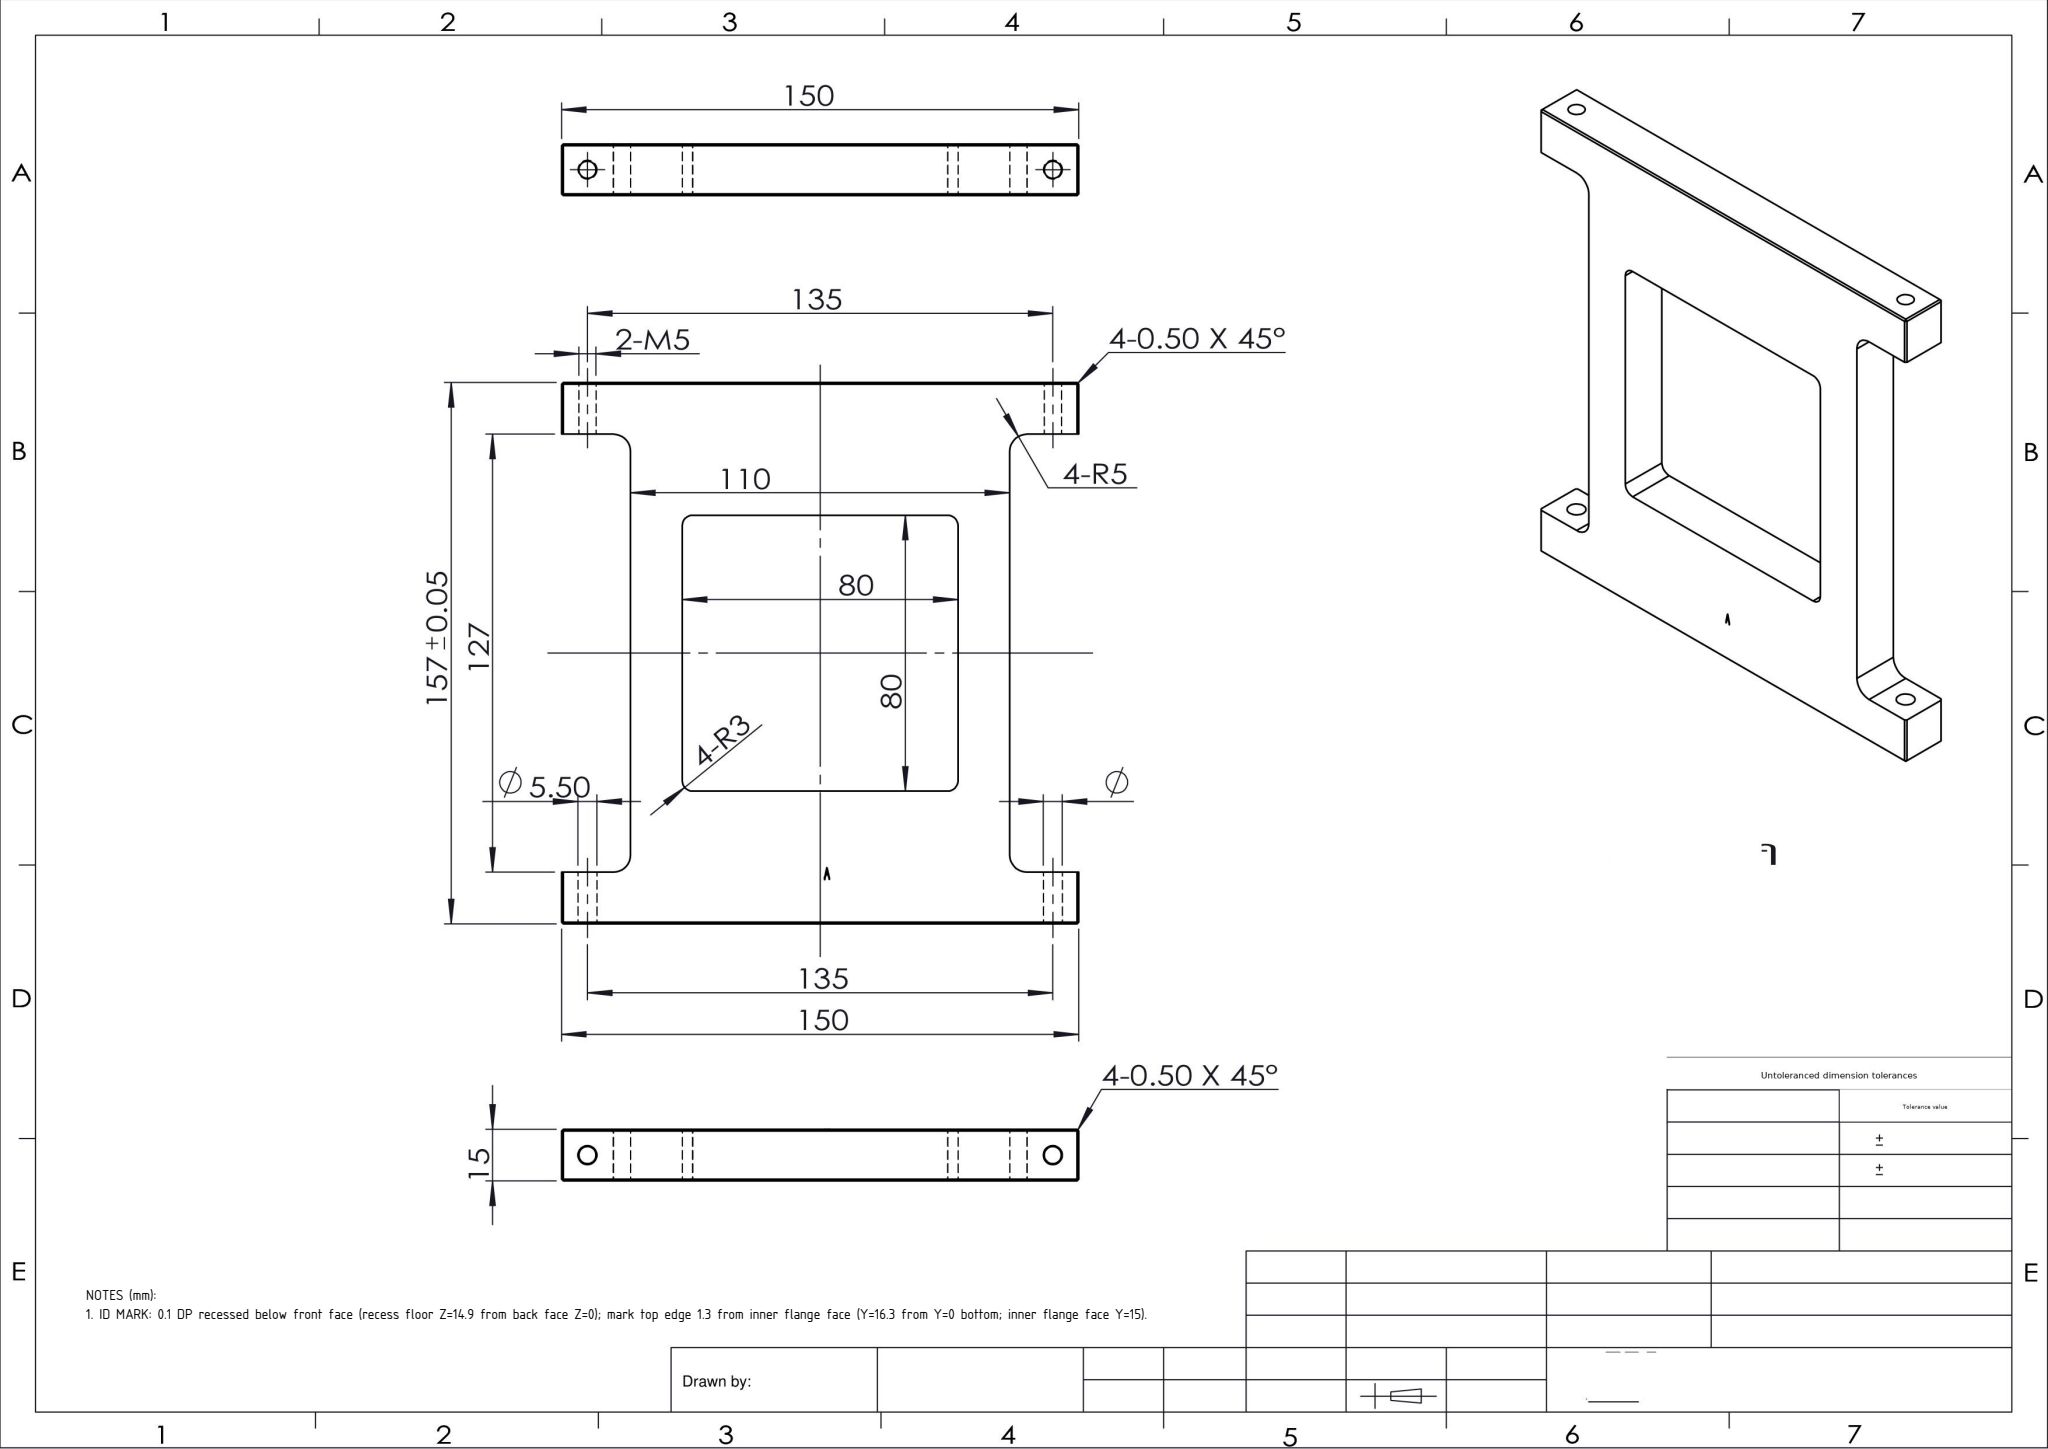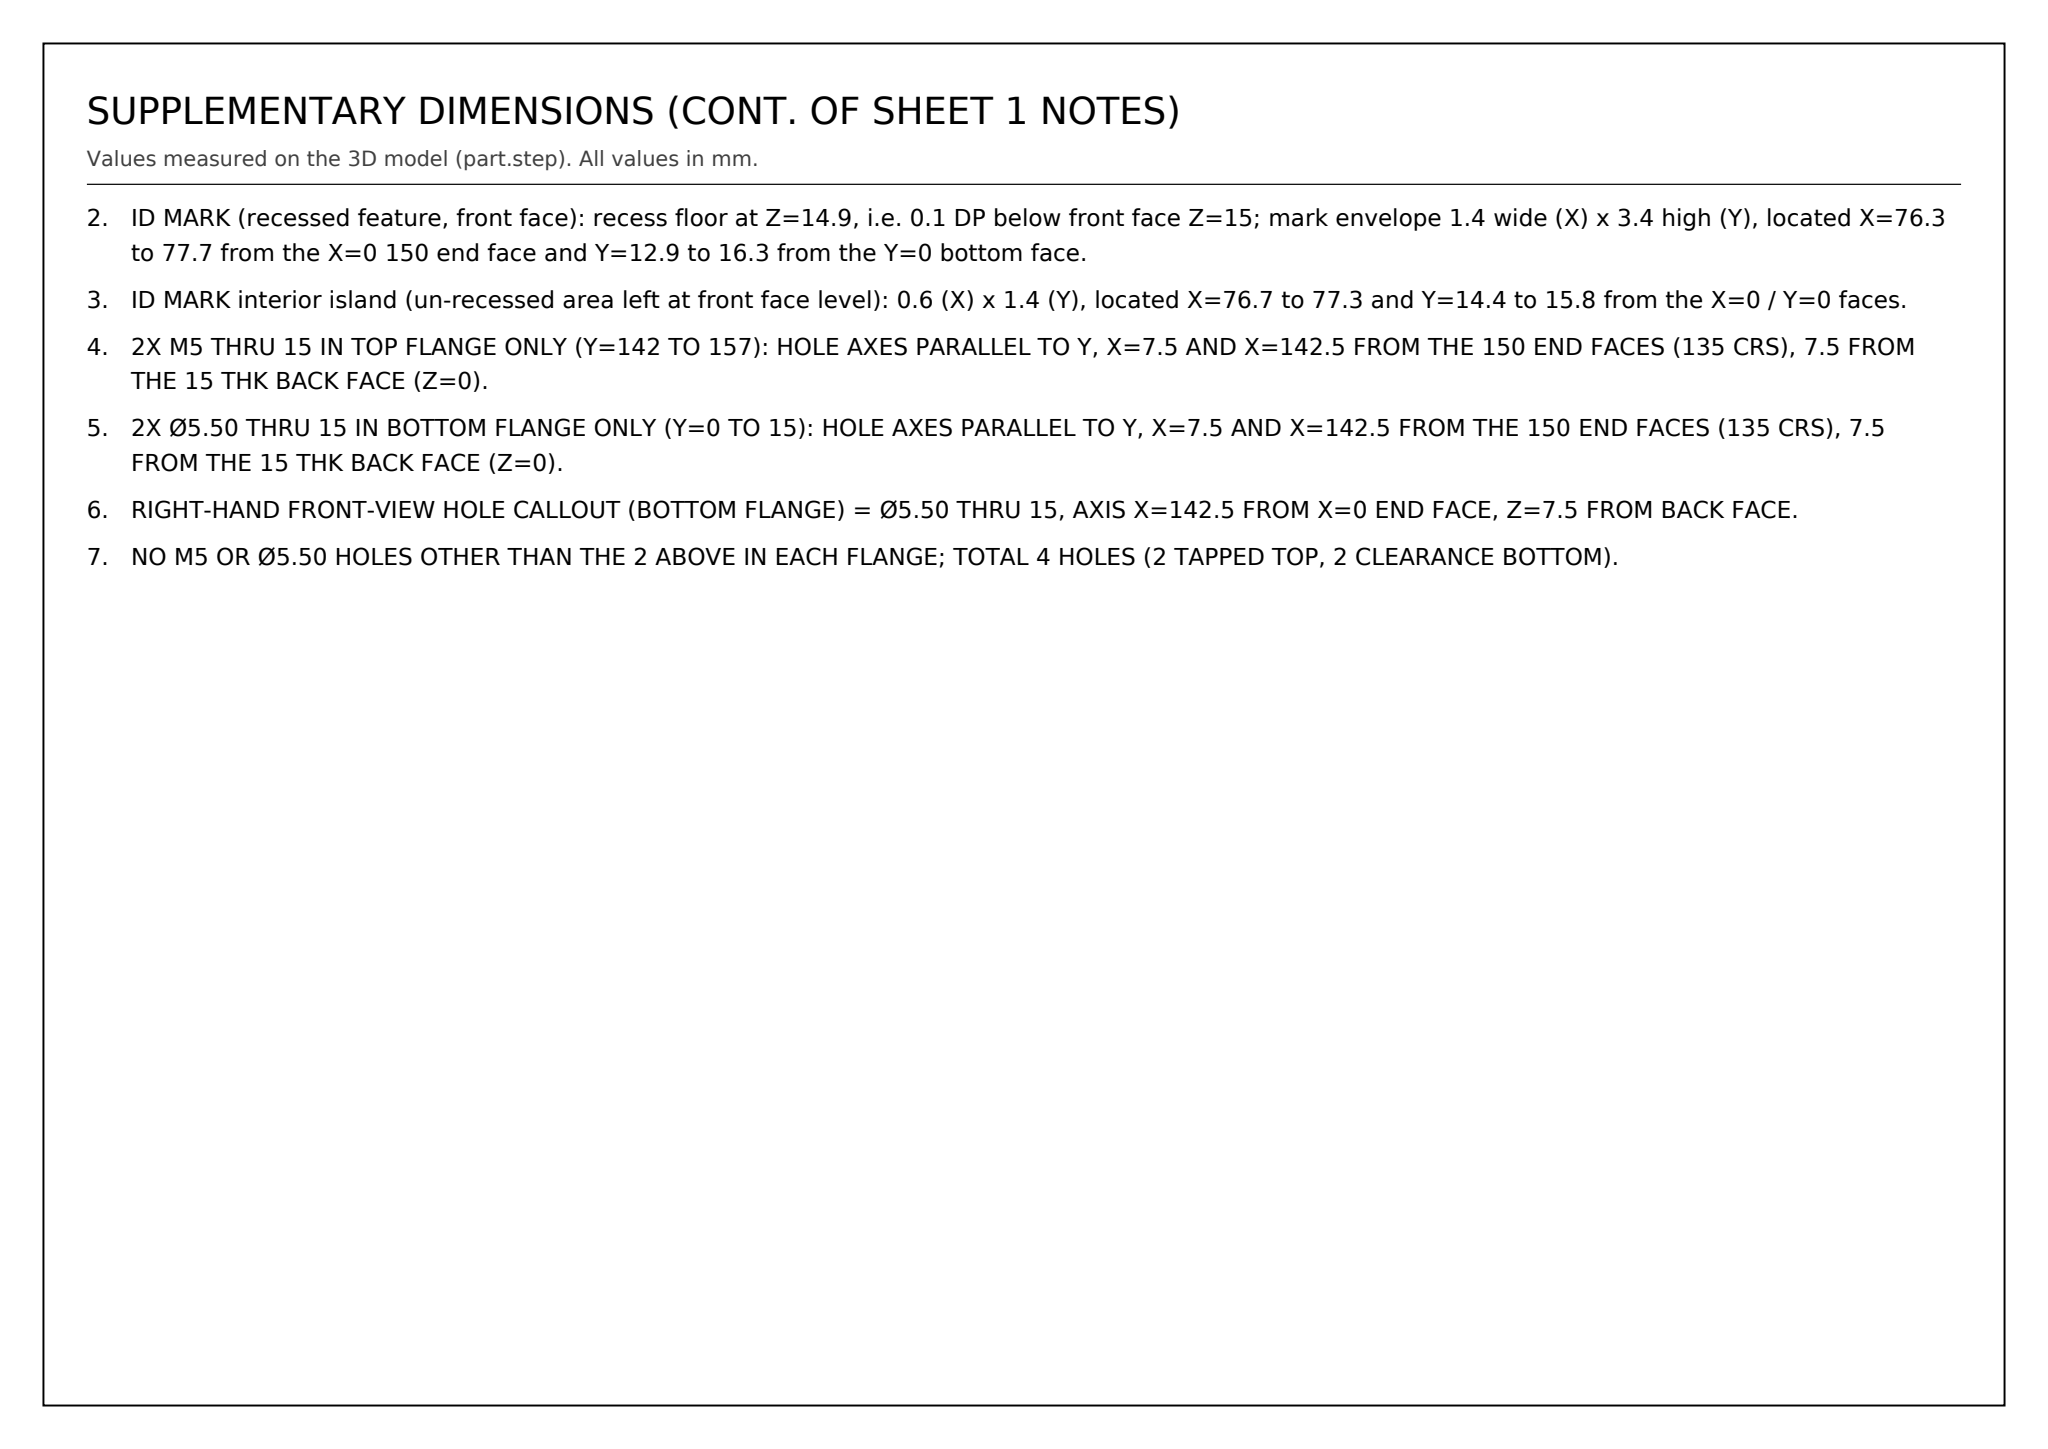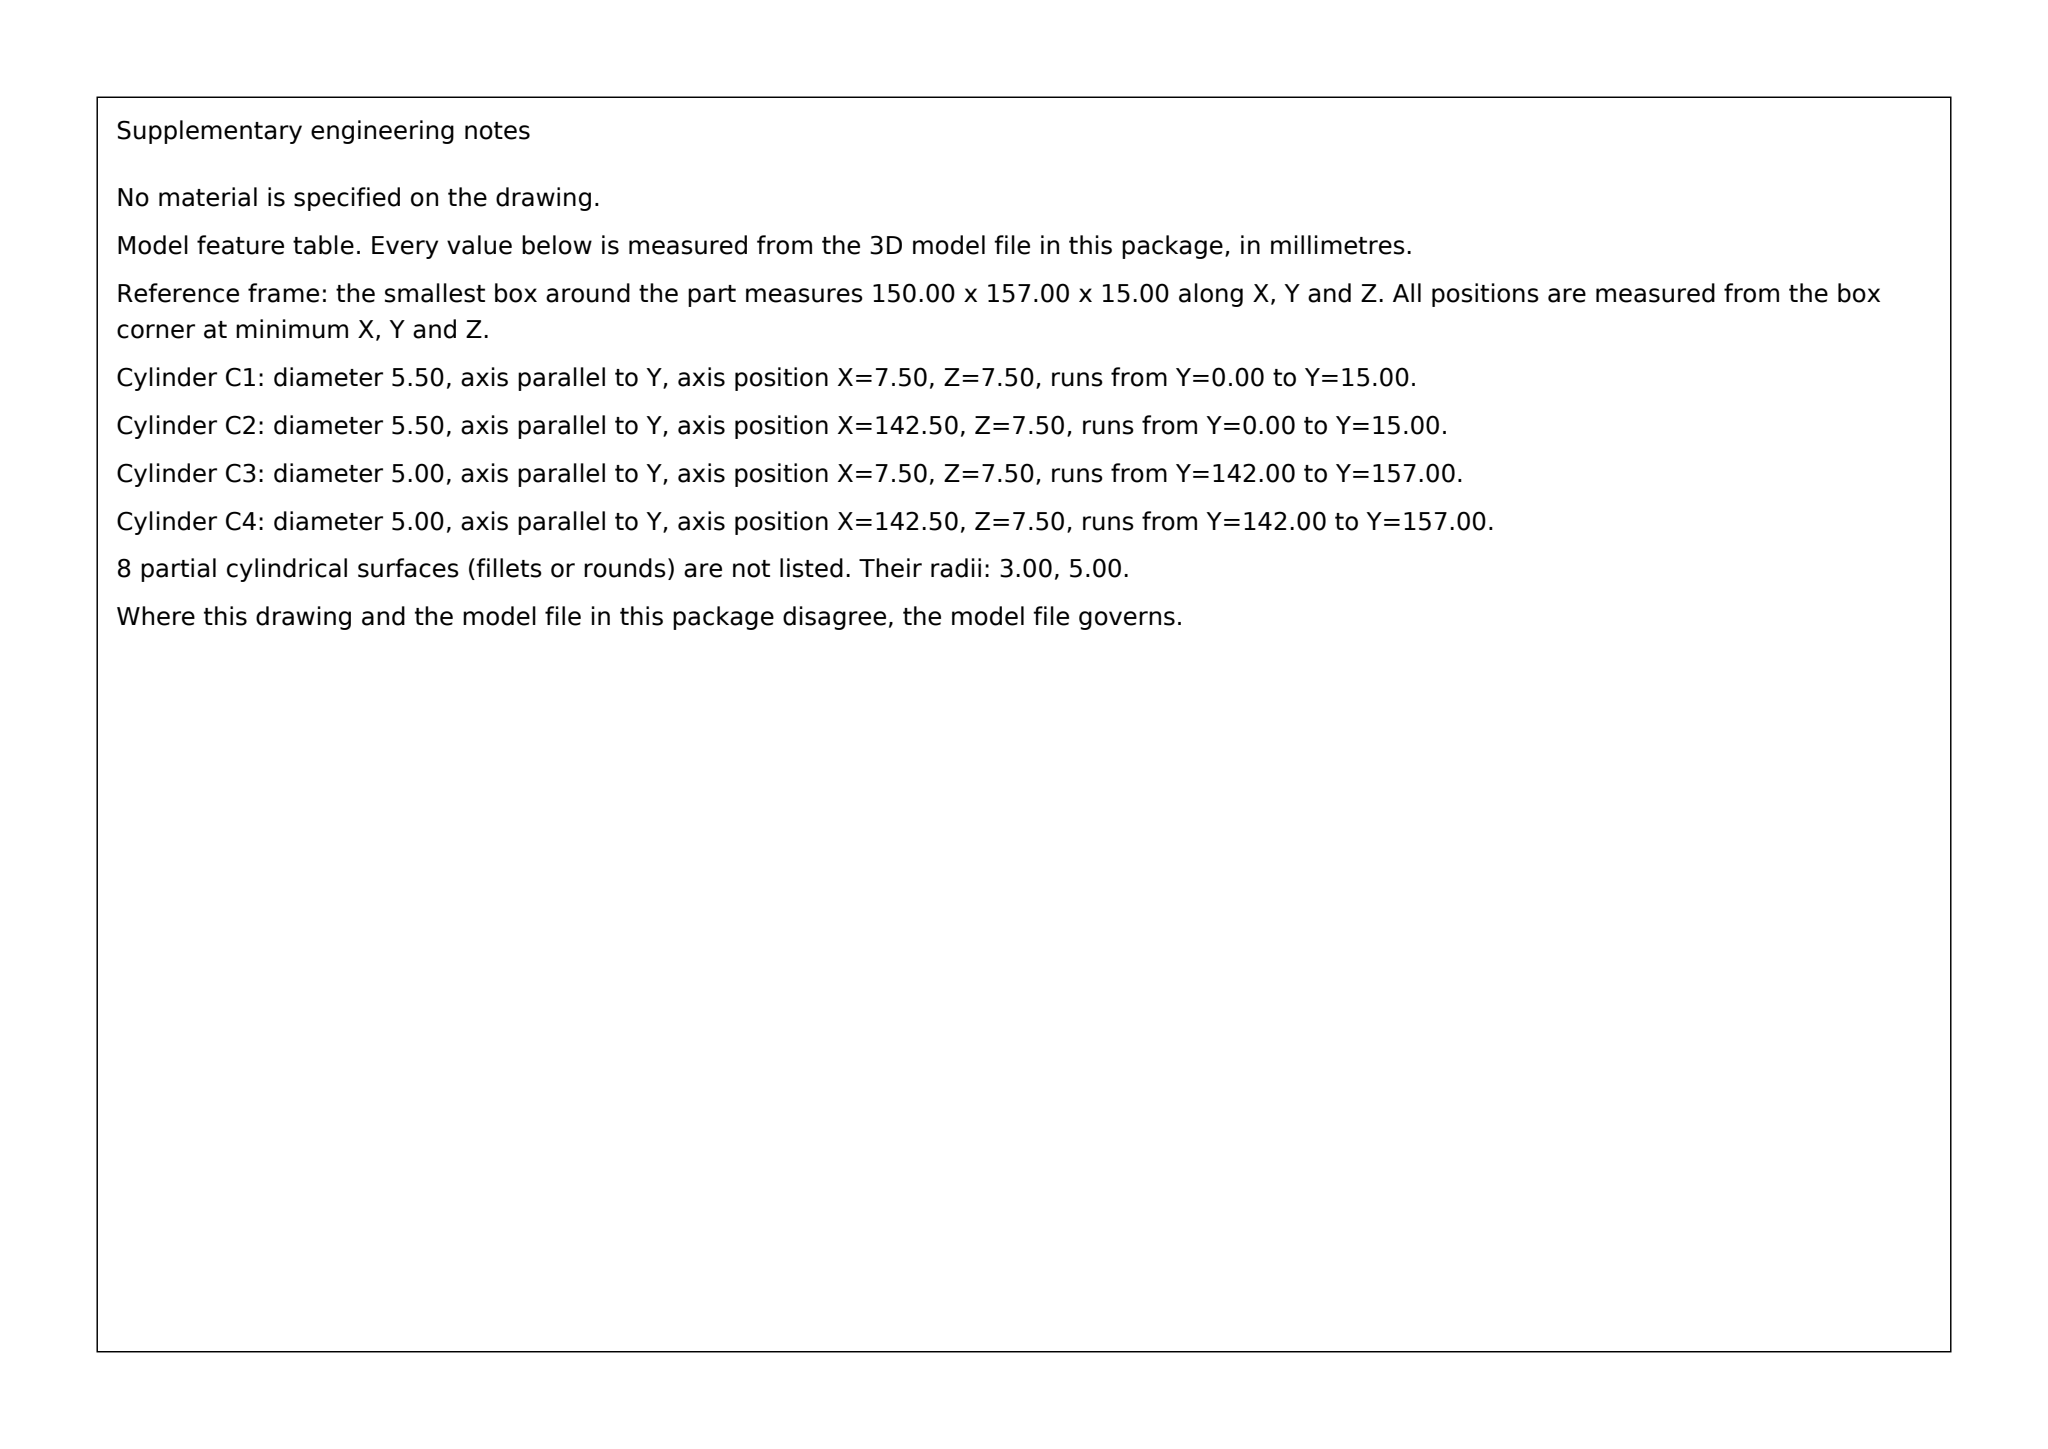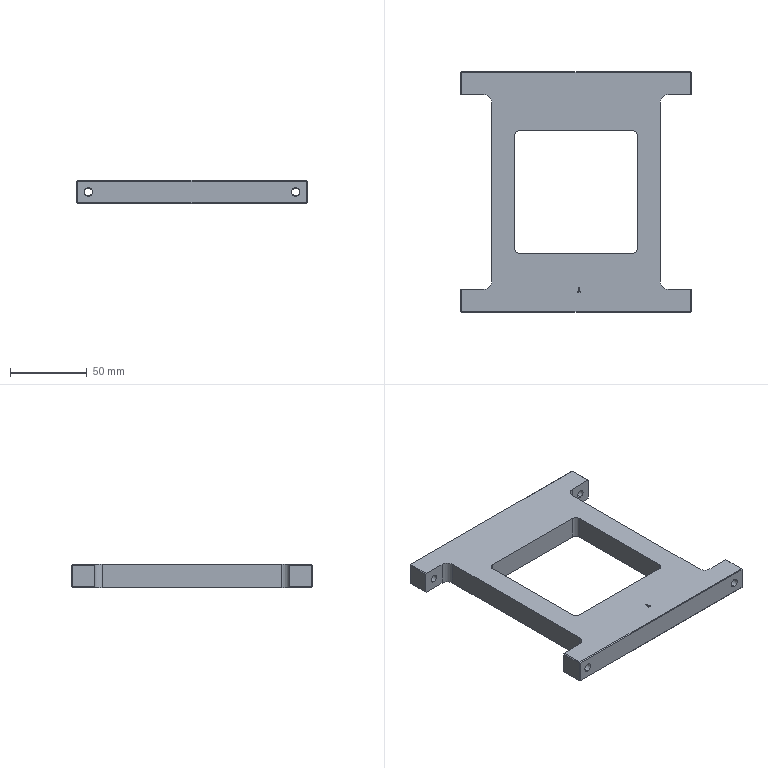Part | SolidWorks | mm | 1 solid | 86 faces | box 150 x 157 x 15 mm | volume 180089 mm3 | plane 63 | cylinder 16 | spline 7 | commonest cylinder face diameters 5.5 x4 5 x4 10 x4 6 x4
Drawing notes:
ID MARK: 0.1 DP recessed below front face (recess floor Z=14.9 from back face Z=0); mark top edge 1.3 from inner flange face (Y=16.3 from Y=0 bottom; inner flange face Y=15). | from the solid: axis_planes: z=14.9 plane x[76.3,77.7] y[12.9,16.3] (0.1 below front face z=15.0); y=16.3 plane at x[76.9,77.0], z[14.9,15.0]; flange inner face y=15.0; 16.3-15.0=1.3
ID MARK (recessed feature, front face): recess floor at Z=14.9, i.e. 0.1 DP below front face Z=15; mark envelope 1.4 wide (X) x 3.4 high (Y), located X=76.3 to 77.7 from the X=0 150 end face and Y=12.9 to 16.3 from the Y=0 bottom face. | from the solid: axis_planes[z, offset 14.9, extent x:[76.3,77.7], y:[12.9,16.3]] and axis_planes[z, offset 15.0] front face
ID MARK interior island (un-recessed area left at front face level): 0.6 (X) x 1.4 (Y), located X=76.7 to 77.3 and Y=14.4 to 15.8 from the X=0 / Y=0 faces. | from the solid: axis_planes[z, offset 15.0, extent x:[76.7,77.3], y:[14.4,15.8]]
2X M5 THRU 15 IN TOP FLANGE ONLY (Y=142 TO 157): HOLE AXES PARALLEL TO Y, X=7.5 AND X=142.5 FROM THE 150 END FACES (135 CRS), 7.5 FROM THE 15 THK BACK FACE (Z=0). | from the solid: cylinders: hole/bore dia 5.0 axis y at (x=7.5,z=7.5) and (x=142.5,z=7.5), from y=142 to y=157
2X Ø5.50 THRU 15 IN BOTTOM FLANGE ONLY (Y=0 TO 15): HOLE AXES PARALLEL TO Y, X=7.5 AND X=142.5 FROM THE 150 END FACES (135 CRS), 7.5 FROM THE 15 THK BACK FACE (Z=0). | from the solid: cylinders: hole/bore dia 5.5 axis y at (x=7.5,z=7.5) and (x=142.5,z=7.5), from y=0 to y=15
RIGHT-HAND FRONT-VIEW HOLE CALLOUT (BOTTOM FLANGE) = Ø5.50 THRU 15, AXIS X=142.5 FROM X=0 END FACE, Z=7.5 FROM BACK FACE. | from the solid: cylinders: hole/bore dia 5.5 axis y at (x=142.5,z=7.5), from y=0 to y=15
NO M5 OR Ø5.50 HOLES OTHER THAN THE 2 ABOVE IN EACH FLANGE; TOTAL 4 HOLES (2 TAPPED TOP, 2 CLEARANCE BOTTOM). | from the solid: cylinders list contains only 4 full 360° hole/bore entries (2X dia 5.0, 2X dia 5.5)
build123d program:
from build123d import *

# Parameters (mm, degrees)
SKETCH1_W           = 150
SKETCH1_H           = 157
BOSS_EXTRUDE1_DEPTH = 7.5
SKETCH2_R           = 2.5
CUT_EXTRUDE1_DEPTH  = 20
SKETCH3_W           = 20
SKETCH3_H           = 127
CUT_EXTRUDE2_DEPTH  = 110.6
FILLET1_R           = 5
CHAMFER1_SIZE       = 0.5
SKETCH5_W           = 80
SKETCH5_H           = 80
CUT_EXTRUDE4_DEPTH  = 110.6
FILLET2_R           = 3
CUT_EXTRUDE5_DEPTH  = 0.1
SKETCH7_R           = 2.75
CUT_EXTRUDE6_DEPTH  = 20


with BuildPart() as part:
    # Sketch1 → Boss-Extrude1 (new, symmetric)
    with BuildSketch(Plane.XY):
        Rectangle(SKETCH1_W, SKETCH1_H)
    extrude(amount=BOSS_EXTRUDE1_DEPTH, both=True)

    # Sketch2 → Cut-Extrude1 (cut)
    with BuildSketch(Plane(origin=(0, 78.5, 0), x_dir=(1, 0, 0), z_dir=(0, 1, 0))):
        with Locations(Location((-67.5, 0, 0), (0, 0, 270))):
            Circle(SKETCH2_R)
        with Locations(Location((67.5, 0, 0), (0, 0, 90))):
            Circle(SKETCH2_R)
    extrude(amount=-CUT_EXTRUDE1_DEPTH, mode=Mode.SUBTRACT)

    # Sketch3 → Cut-Extrude2 (cut, through all)
    with BuildSketch(Plane(origin=(0, 0, -7.5), x_dir=(-1, 0, 0), z_dir=(0, 0, -1))):
        with Locations((-65, 0)):
            Rectangle(SKETCH3_W, SKETCH3_H)
        with Locations((65, 0)):
            Rectangle(SKETCH3_W, SKETCH3_H)
    extrude(amount=-CUT_EXTRUDE2_DEPTH, mode=Mode.SUBTRACT)

    # Fillet1
    fillet1_edges = [part.edges().sort_by_distance(p)[0] for p in [
        (55, 63.5, 0),
        (55, -63.5, 0),
        (-55, 63.5, 0),
        (-55, -63.5, 0),
    ]]
    fillet(fillet1_edges, radius=FILLET1_R)

    # Chamfer1
    chamfer1_edges = [part.edges().sort_by_distance(p)[0] for p in [
        (-75, 71, 7.5),
        (0, -78.5, 7.5),
        (75, 71, -7.5),
        (75, 71, 7.5),
        (-75, -71, -7.5),
        (-75, -71, 7.5),
        (75, -71, 7.5),
        (0, -78.5, -7.5),
        (-75, 71, -7.5),
        (0, 78.5, -7.5),
        (75, -71, -7.5),
        (0, 78.5, 7.5),
        (75, -78.5, 0),
        (-75, -78.5, 0),
        (-75, 78.5, 0),
        (75, 78.5, 0),
    ]]
    chamfer(chamfer1_edges, length=CHAMFER1_SIZE)

    # Sketch5 → Cut-Extrude4 (cut, through all)
    with BuildSketch(Plane.XY.offset(7.5)):
        Rectangle(SKETCH5_W, SKETCH5_H)
    extrude(amount=-CUT_EXTRUDE4_DEPTH, mode=Mode.SUBTRACT)

    # Fillet2
    fillet2_edges = [part.edges().sort_by_distance(p)[0] for p in [
        (-40, -40, 0),
        (-40, 40, 0),
        (40, 40, 0),
        (40, -40, 0),
    ]]
    fillet(fillet2_edges, radius=FILLET2_R)

    # Sketch6 → Cut-Extrude5 (cut)
    with BuildSketch(Plane.XY.offset(7.5)):
        with BuildLine():
            Line((2.312, -64.158), (1.627, -64.324))
            Line((1.627, -64.324), (1.466, -65.074))
            Line((1.466, -65.074), (1.39, -65.457))
            Line((1.39, -65.457), (1.36, -65.578))
            add(Edge.make_bspline(
                [(1.36, -65.578), (1.357, -65.586), (1.352, -65.601), (1.342, -65.618), (1.331, -65.626), (1.318, -65.628), (1.309, -65.617), (1.304, -65.604), (1.302, -65.584), (1.297, -65.558), (1.295, -65.521), (1.291, -65.493), (1.289, -65.477)],
                knots=[0, 0, 0, 0, 1.227, 2.069, 2.596, 3.064, 3.56, 4.322, 5.03, 6.209, 7.852, 10, 10, 10, 10], degree=3))
            Line((1.289, -65.477), (1.265, -65.266))
            add(Edge.make_bspline(
                [(1.265, -65.266), (1.263, -65.249), (1.26, -65.218), (1.258, -65.176), (1.258, -65.147), (1.259, -65.122), (1.267, -65.099), (1.275, -65.083), (1.28, -65.074)],
                knots=[0, 0, 0, 0, 1.604, 2.861, 3.774, 4.323, 5.132, 6, 6, 6, 6], degree=3))
            Line((1.28, -65.074), (1.305, -65.029))
            add(Edge.make_bspline(
                [(1.305, -65.029), (1.311, -65.017), (1.324, -64.989), (1.34, -64.937), (1.357, -64.869), (1.375, -64.791), (1.392, -64.715), (1.406, -64.653), (1.417, -64.613), (1.424, -64.592), (1.426, -64.586)],
                knots=[0, 0, 0, 0, 0.6797, 1.623, 2.844, 4.336, 5.799, 6.891, 7.631, 8, 8, 8, 8], degree=3))
            Line((1.426, -64.586), (1.944, -62.185))
            Line((1.944, -62.185), (2.014, -62.185))
            Line((2.014, -62.185), (2.503, -64.344))
            Line((2.503, -64.344), (2.563, -64.596))
            add(Edge.make_bspline(
                [(2.563, -64.596), (2.569, -64.625), (2.58, -64.676), (2.597, -64.743), (2.61, -64.794), (2.62, -64.821), (2.624, -64.833)],
                knots=[0, 0, 0, 0, 1.426, 2.558, 3.42, 4, 4, 4, 4], degree=3))
            Line((2.624, -64.833), (2.659, -64.928))
            add(Edge.make_bspline(
                [(2.659, -64.928), (2.663, -64.942), (2.67, -64.968), (2.683, -65.001), (2.695, -65.027), (2.711, -65.049), (2.727, -65.066), (2.738, -65.083), (2.739, -65.099), (2.737, -65.113), (2.735, -65.132), (2.734, -65.155), (2.731, -65.188), (2.73, -65.212), (2.73, -65.226)],
                knots=[0, 0, 0, 0, 1.645, 2.997, 4.066, 4.893, 6.03, 6.671, 7.125, 7.802, 8.339, 9.24, 10.452, 12, 12, 12, 12], degree=3))
            Line((2.73, -65.226), (2.709, -65.452))
            Line((2.709, -65.452), (2.699, -65.537))
            add(Edge.make_bspline(
                [(2.699, -65.537), (2.699, -65.547), (2.698, -65.564), (2.693, -65.587), (2.691, -65.603), (2.685, -65.615), (2.674, -65.62), (2.66, -65.616), (2.649, -65.602), (2.646, -65.59), (2.644, -65.583)],
                knots=[0, 0, 0, 0, 1.663, 2.956, 3.874, 4.465, 5.131, 5.832, 6.736, 8, 8, 8, 8], degree=3))
            Line((2.644, -65.583), (2.609, -65.382))
            Line((2.609, -65.382), (2.312, -64.158))
        make_face()
        with BuildLine():
            Line((2.302, -64.082), (1.979, -62.668))
            Line((1.979, -62.668), (1.652, -64.148))
            add(Edge.make_bspline(
                [(1.652, -64.148), (1.68, -64.144), (1.729, -64.136), (1.798, -64.121), (1.862, -64.103), (1.92, -64.087), (1.967, -64.071), (1.998, -64.061), (2.022, -64.05), (2.034, -64.041), (2.04, -64.038)],
                knots=[0, 0, 0, 0, 1.702, 2.938, 4.141, 5.675, 6.466, 7.109, 7.616, 8, 8, 8, 8], degree=3))
            Line((2.04, -64.038), (2.166, -63.952))
            Line((2.166, -63.952), (2.302, -64.082))
        make_face(mode=Mode.SUBTRACT)
    extrude(amount=-CUT_EXTRUDE5_DEPTH, mode=Mode.SUBTRACT)

    # Sketch7 → Cut-Extrude6 (cut)
    with BuildSketch(Plane(origin=(0, -78.5, 0), x_dir=(-1, 0, 0), z_dir=(0, -1, 0))):
        with Locations(Location((67.5, 0, 0), (0, 0, 90))):
            Circle(SKETCH7_R)
        with Locations(Location((-67.5, 0, 0), (0, 0, 90))):
            Circle(SKETCH7_R)
    extrude(amount=-CUT_EXTRUDE6_DEPTH, mode=Mode.SUBTRACT)


solid = part.part